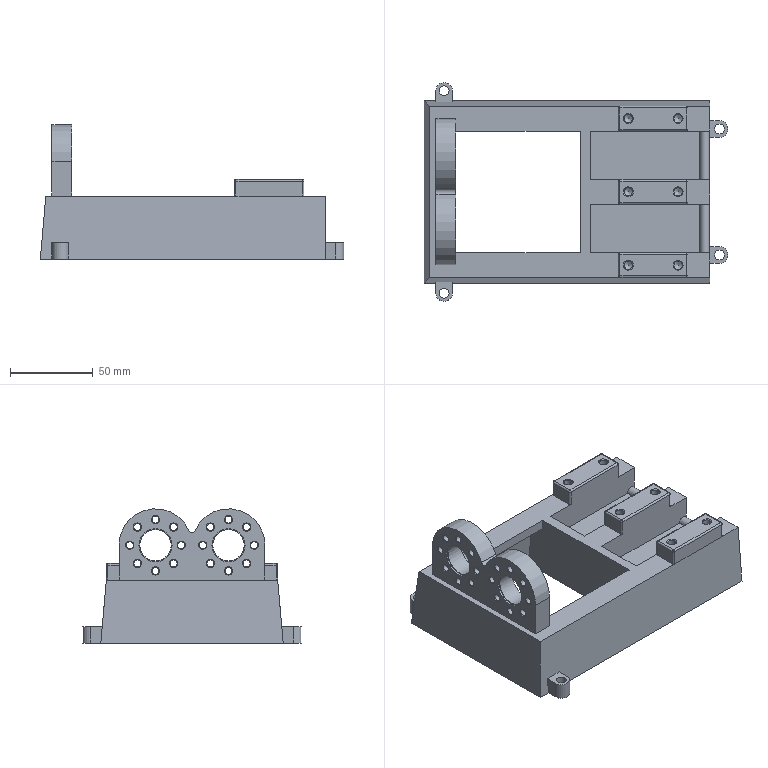Component | NX | BASE | 1 solid | 177 faces | volume 276963 mm3 | cylinder 63 | plane 58 | cone 44 | sphere 12 | commonest cylinder face diameters 2 x24 4.2 x16 6 x6 5 x6 10 x4 19 x2 44 x2 20 x2